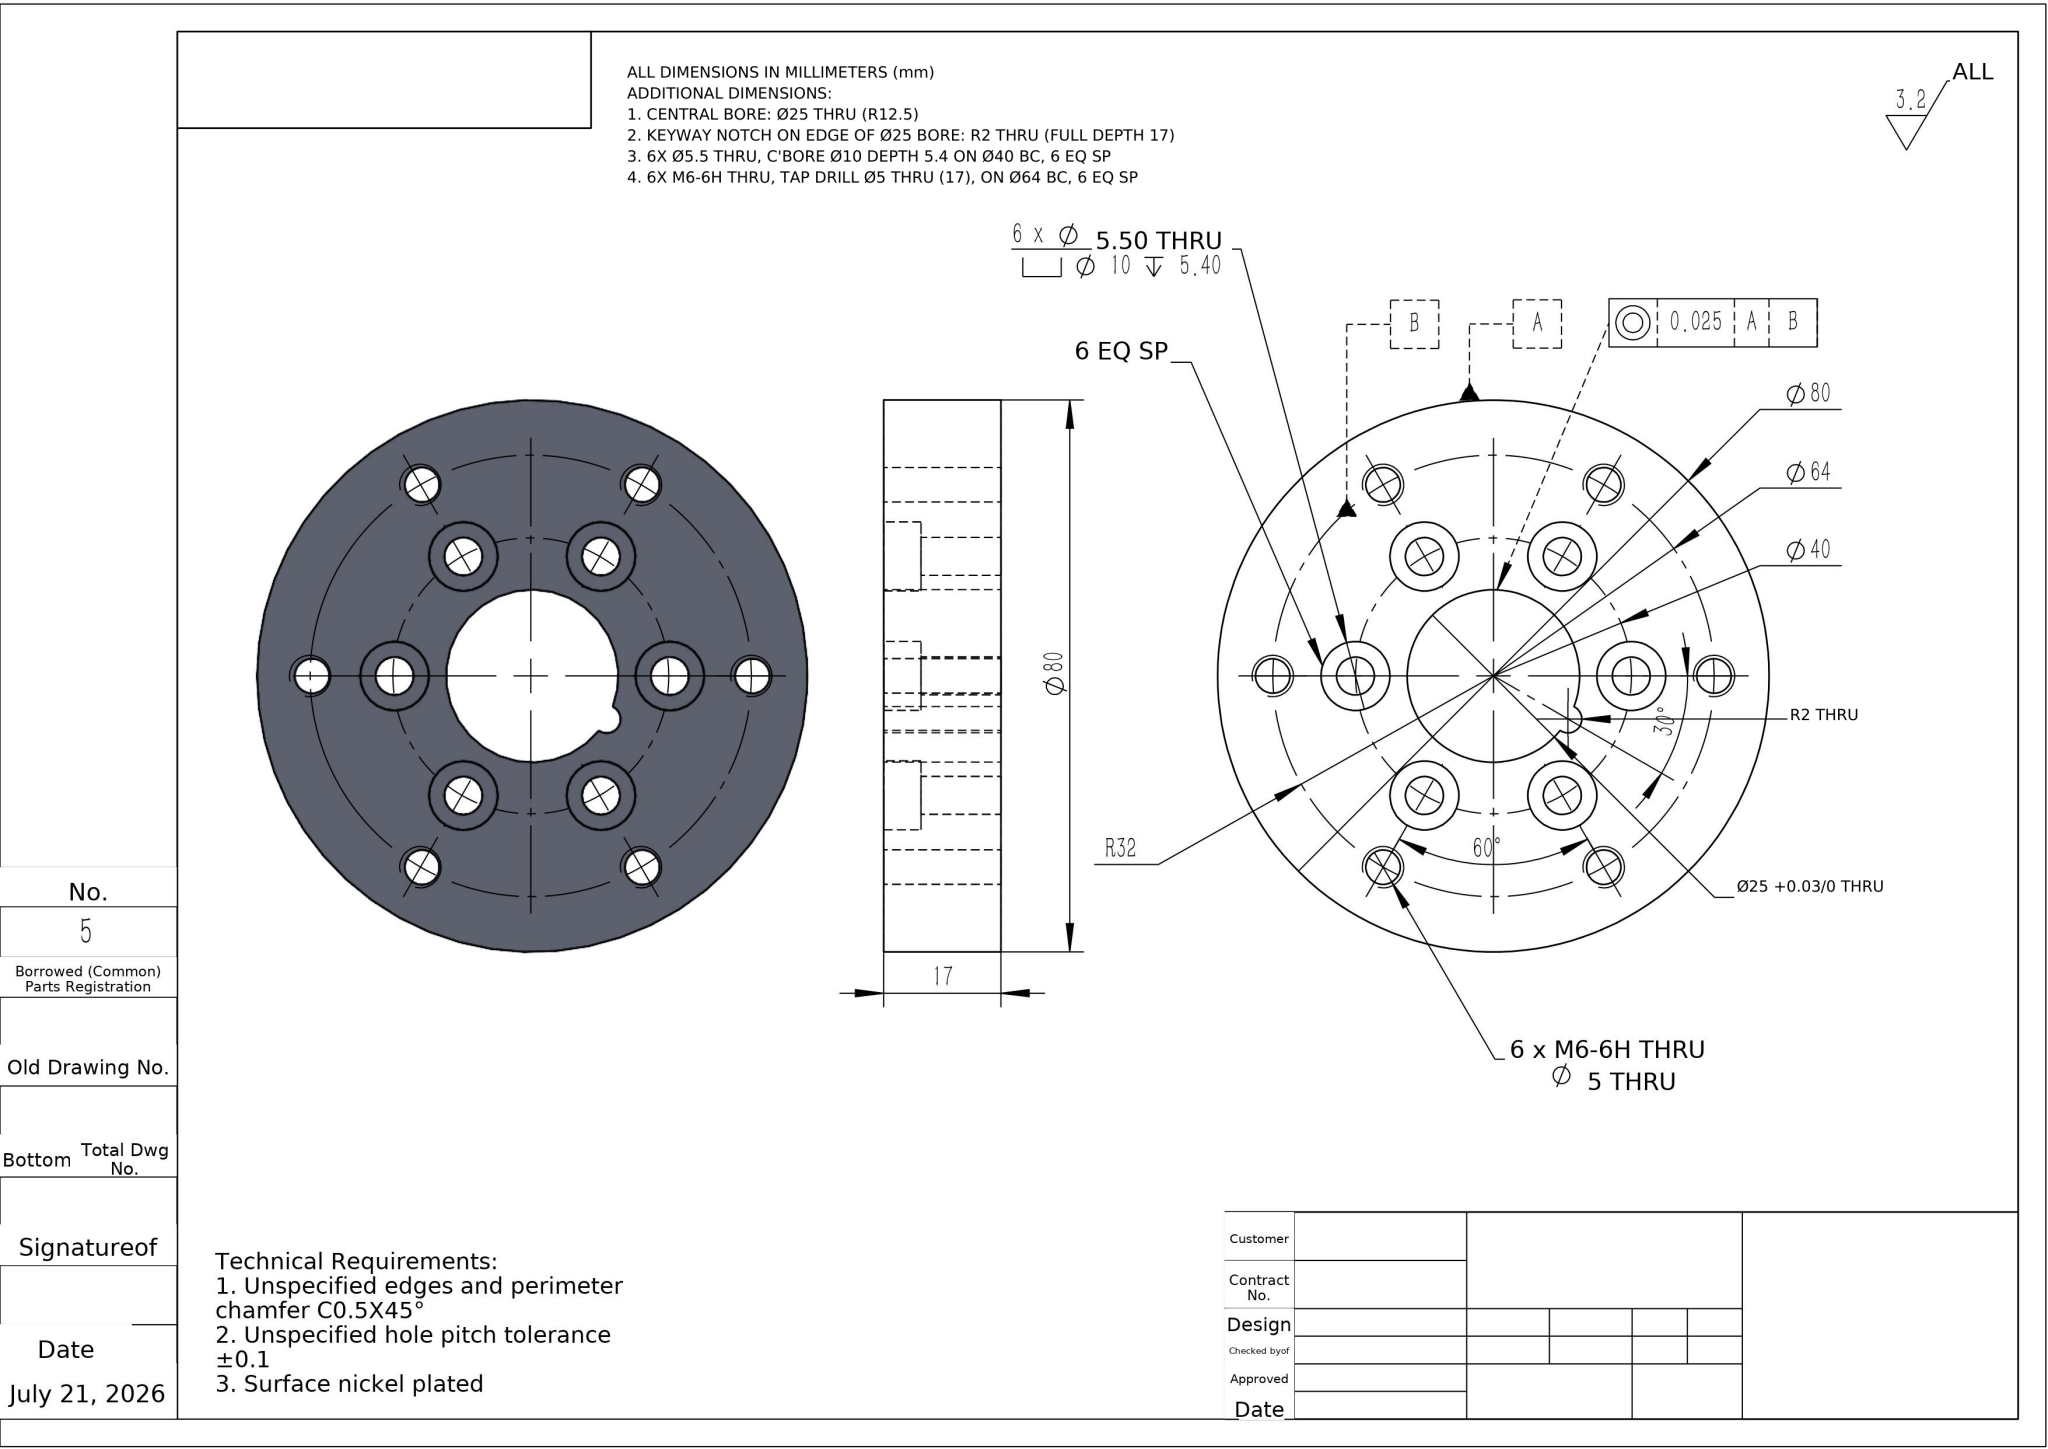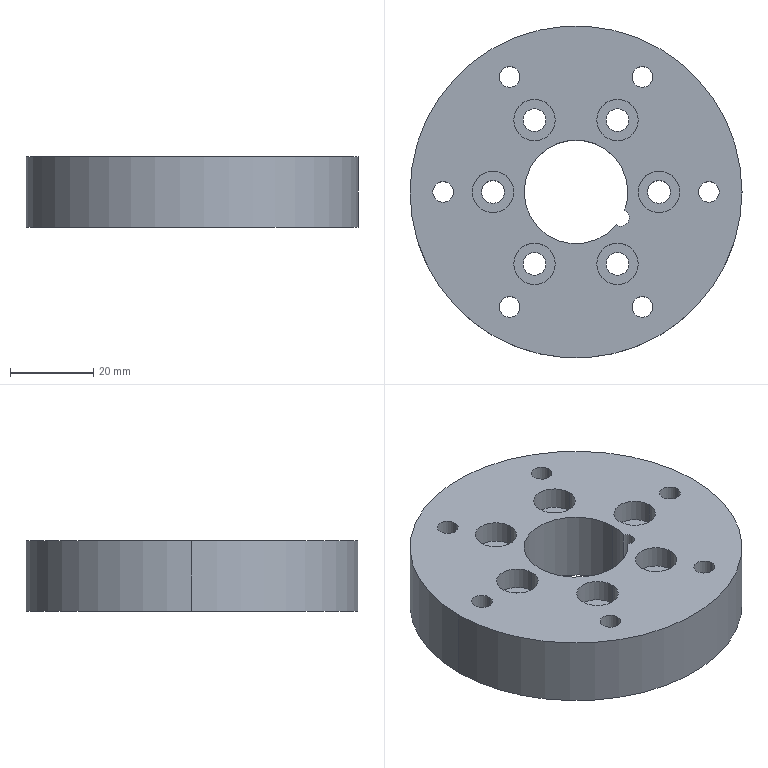Part | NX | mm | 1 solid | 50 faces | box 80 x 80 x 17 mm | volume 70795 mm3 | cylinder 42 | plane 8 | commonest cylinder face diameters 5 x12 10 x12 5.5 x12 25 x3 80 x2 4 x1